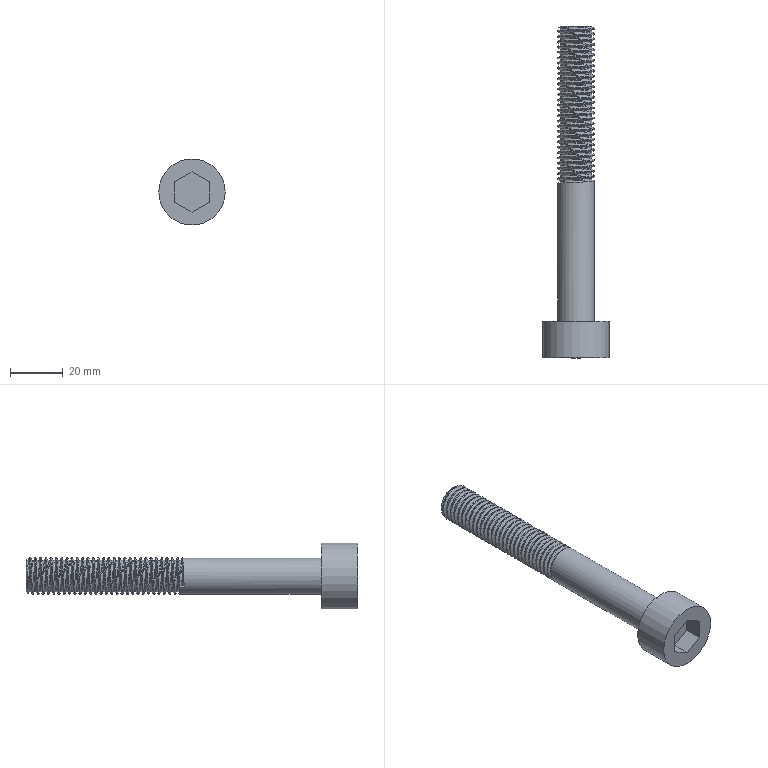Component | NX | ALLINE_SCREW_M14_DP_2_SP | 1 solid | 47 faces | volume 21707 mm3 | cylinder 32 | plane 12 | spline 2 | cone 1 | commonest cylinder face diameters 14 x30 25.2 x1 12 x1